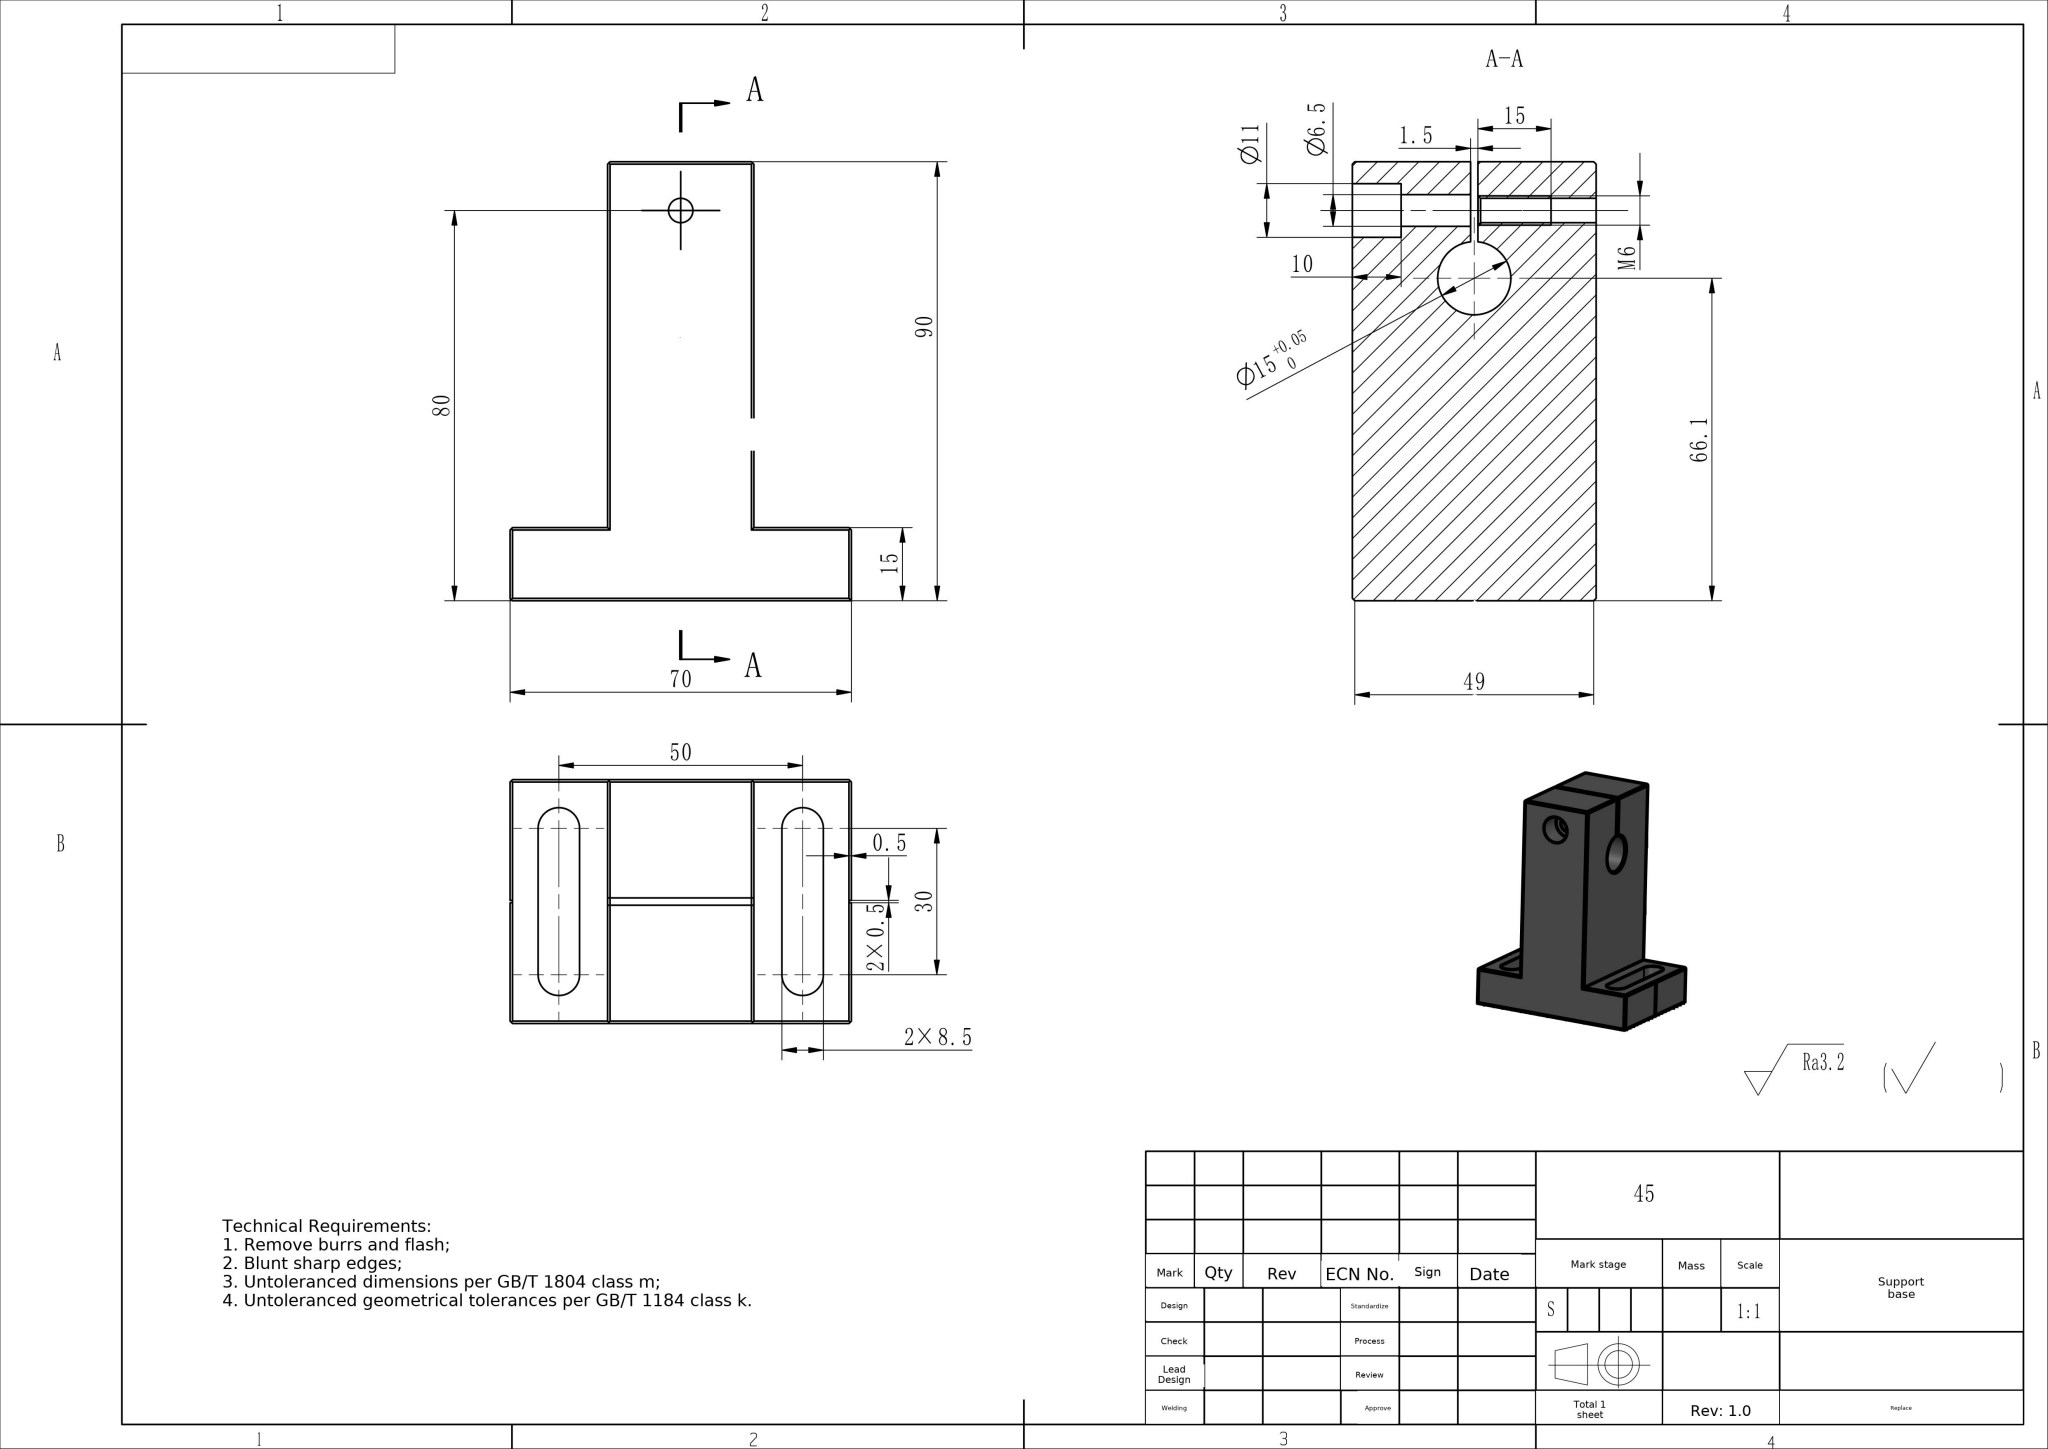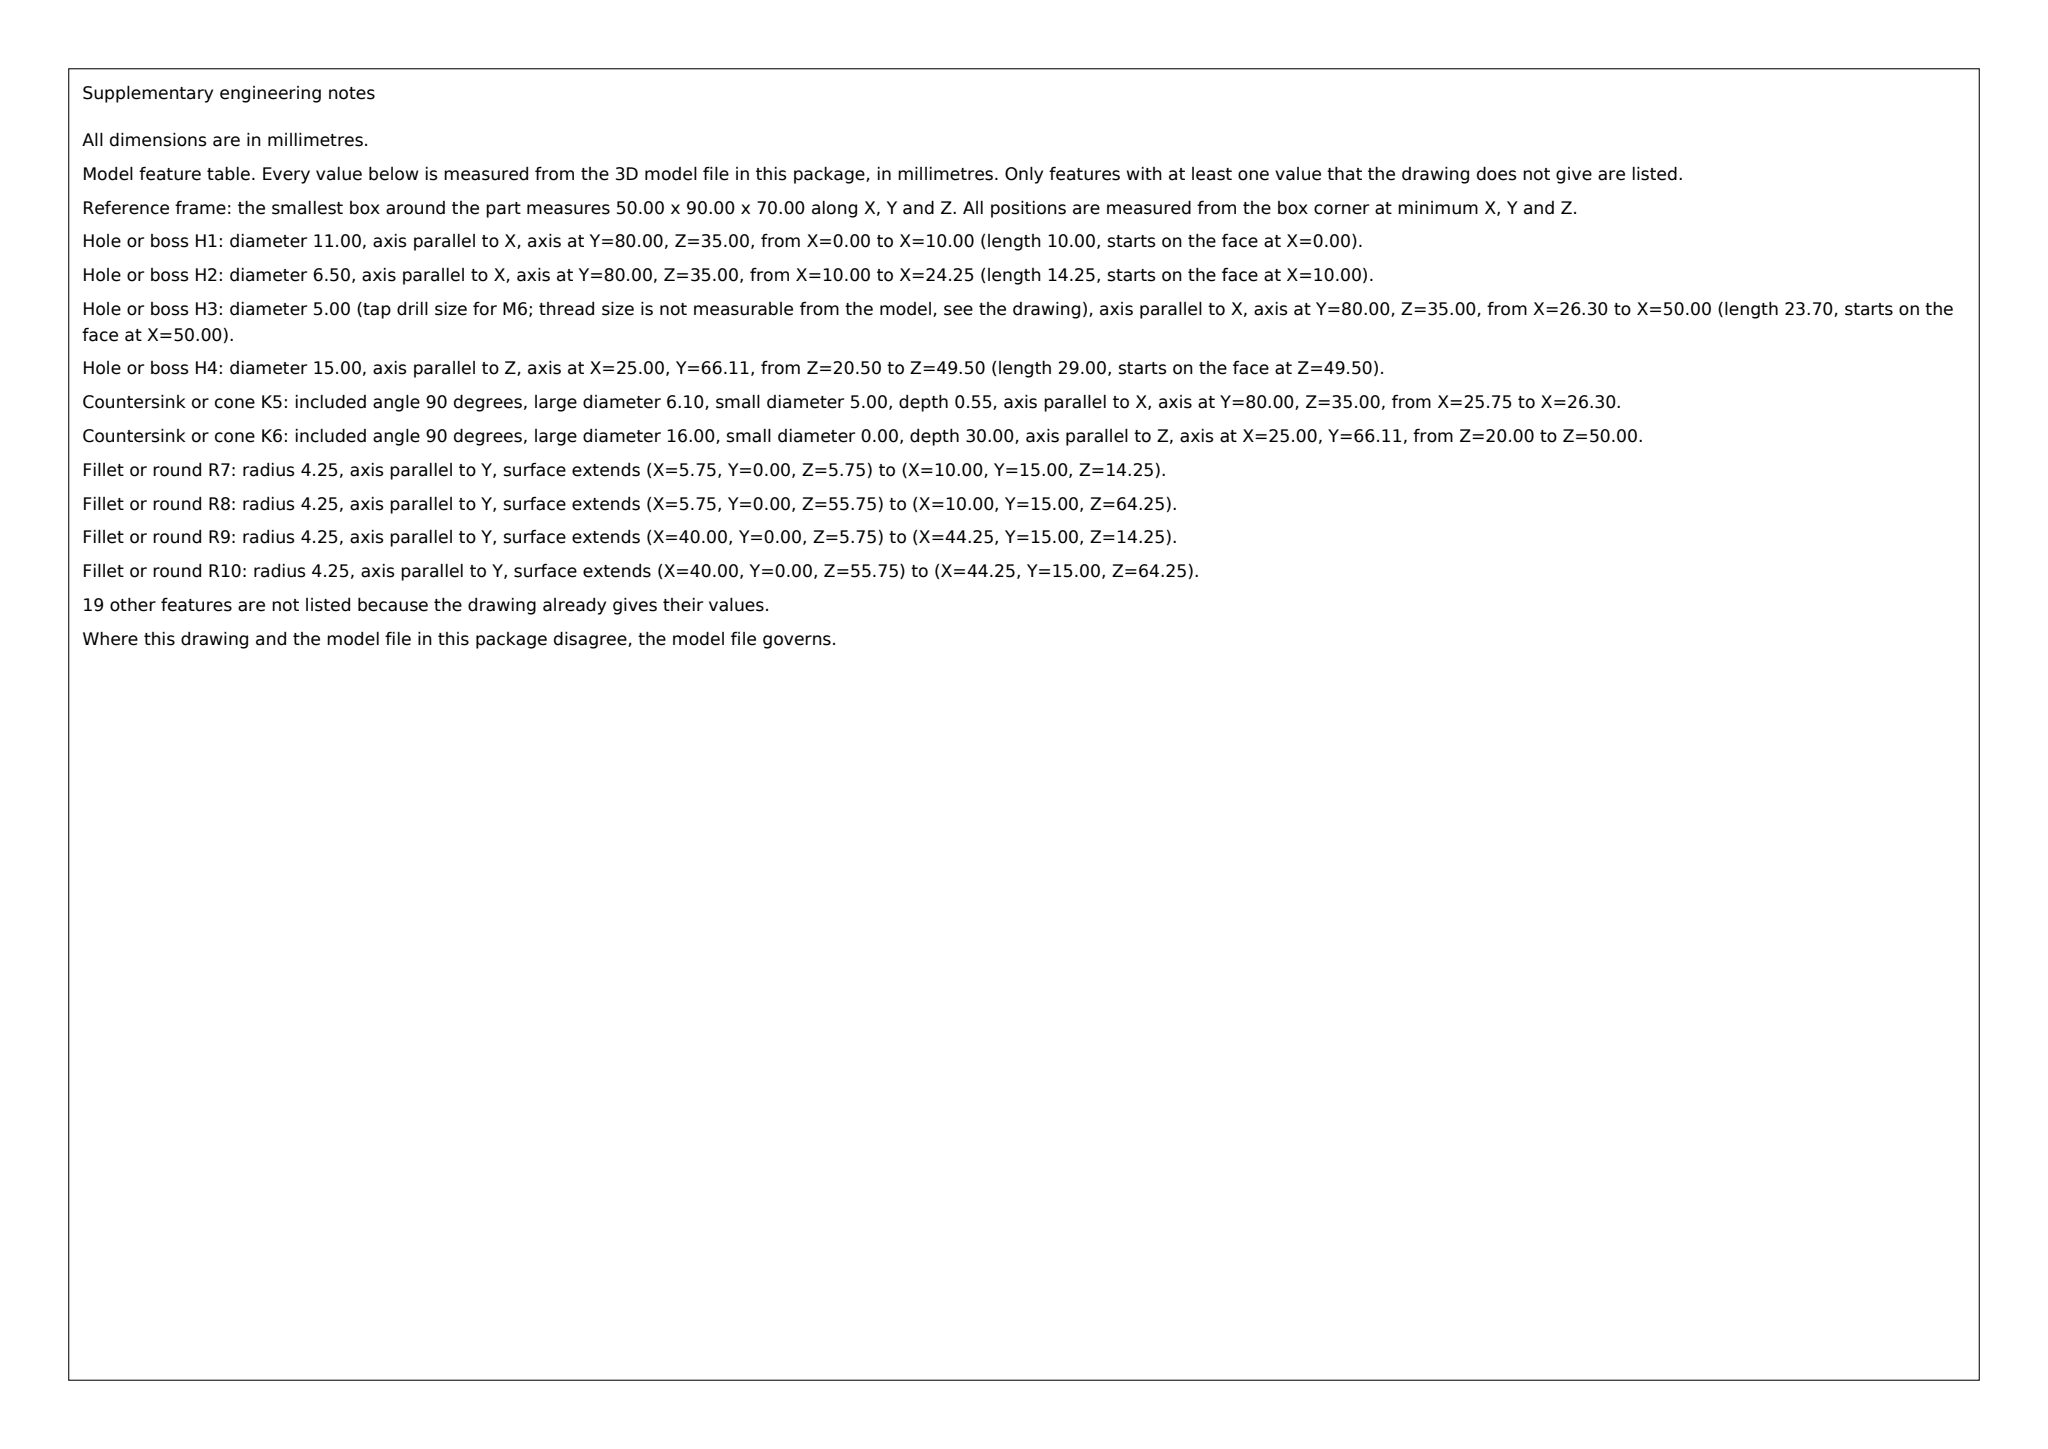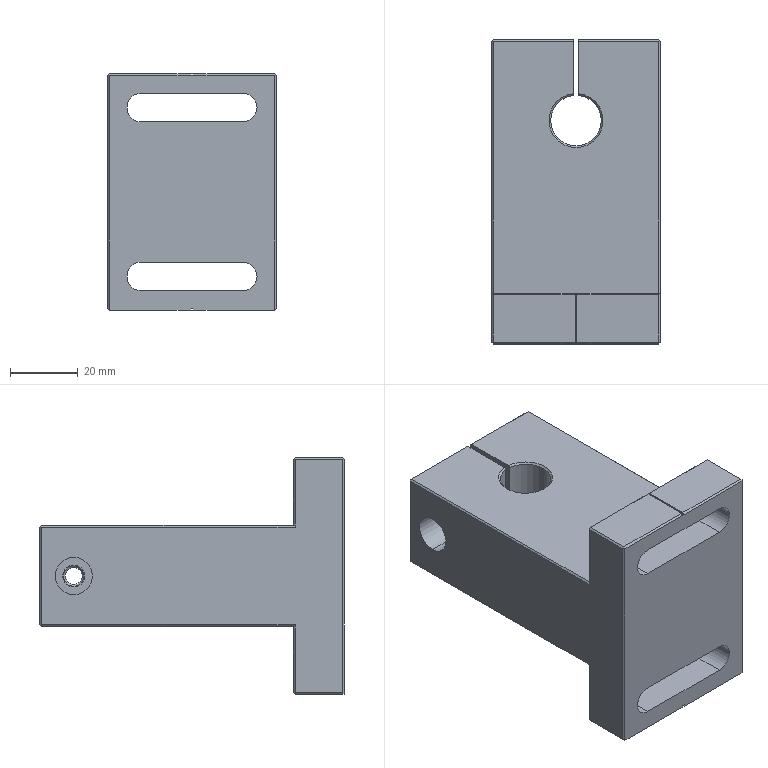Part | SolidWorks | mm | material 45 | 1 solid | 73 faces | box 50 x 90 x 70 mm | volume 147577 mm3 | plane 52 | cylinder 15 | cone 6 | commonest cylinder face diameters 8.5 x6 15 x3 5 x2 6.5 x2 11 x2